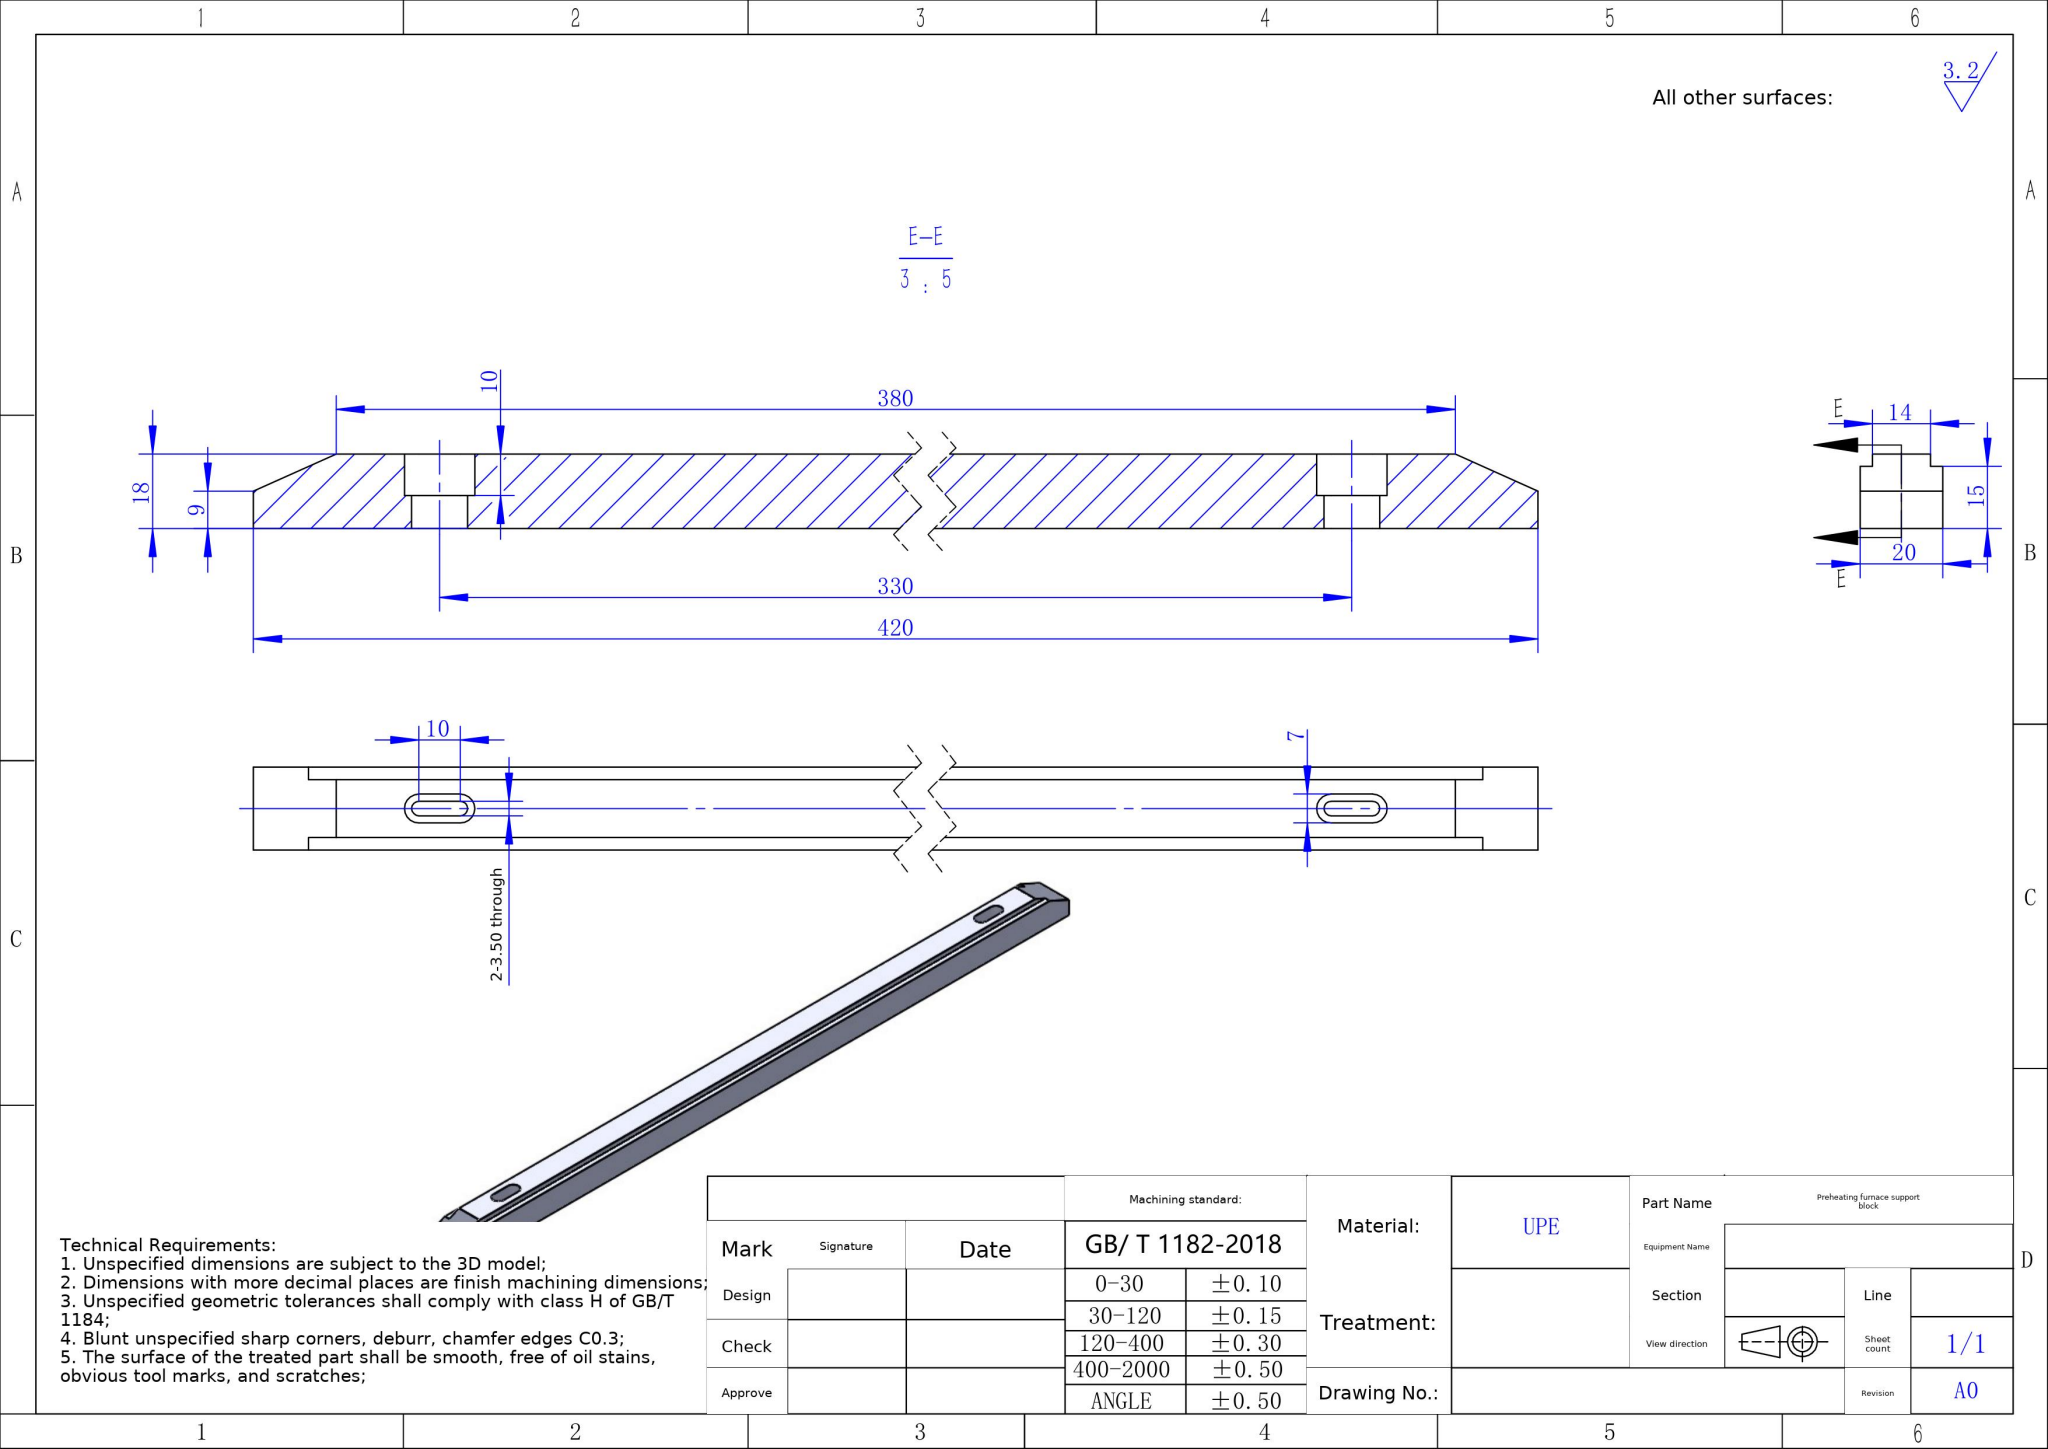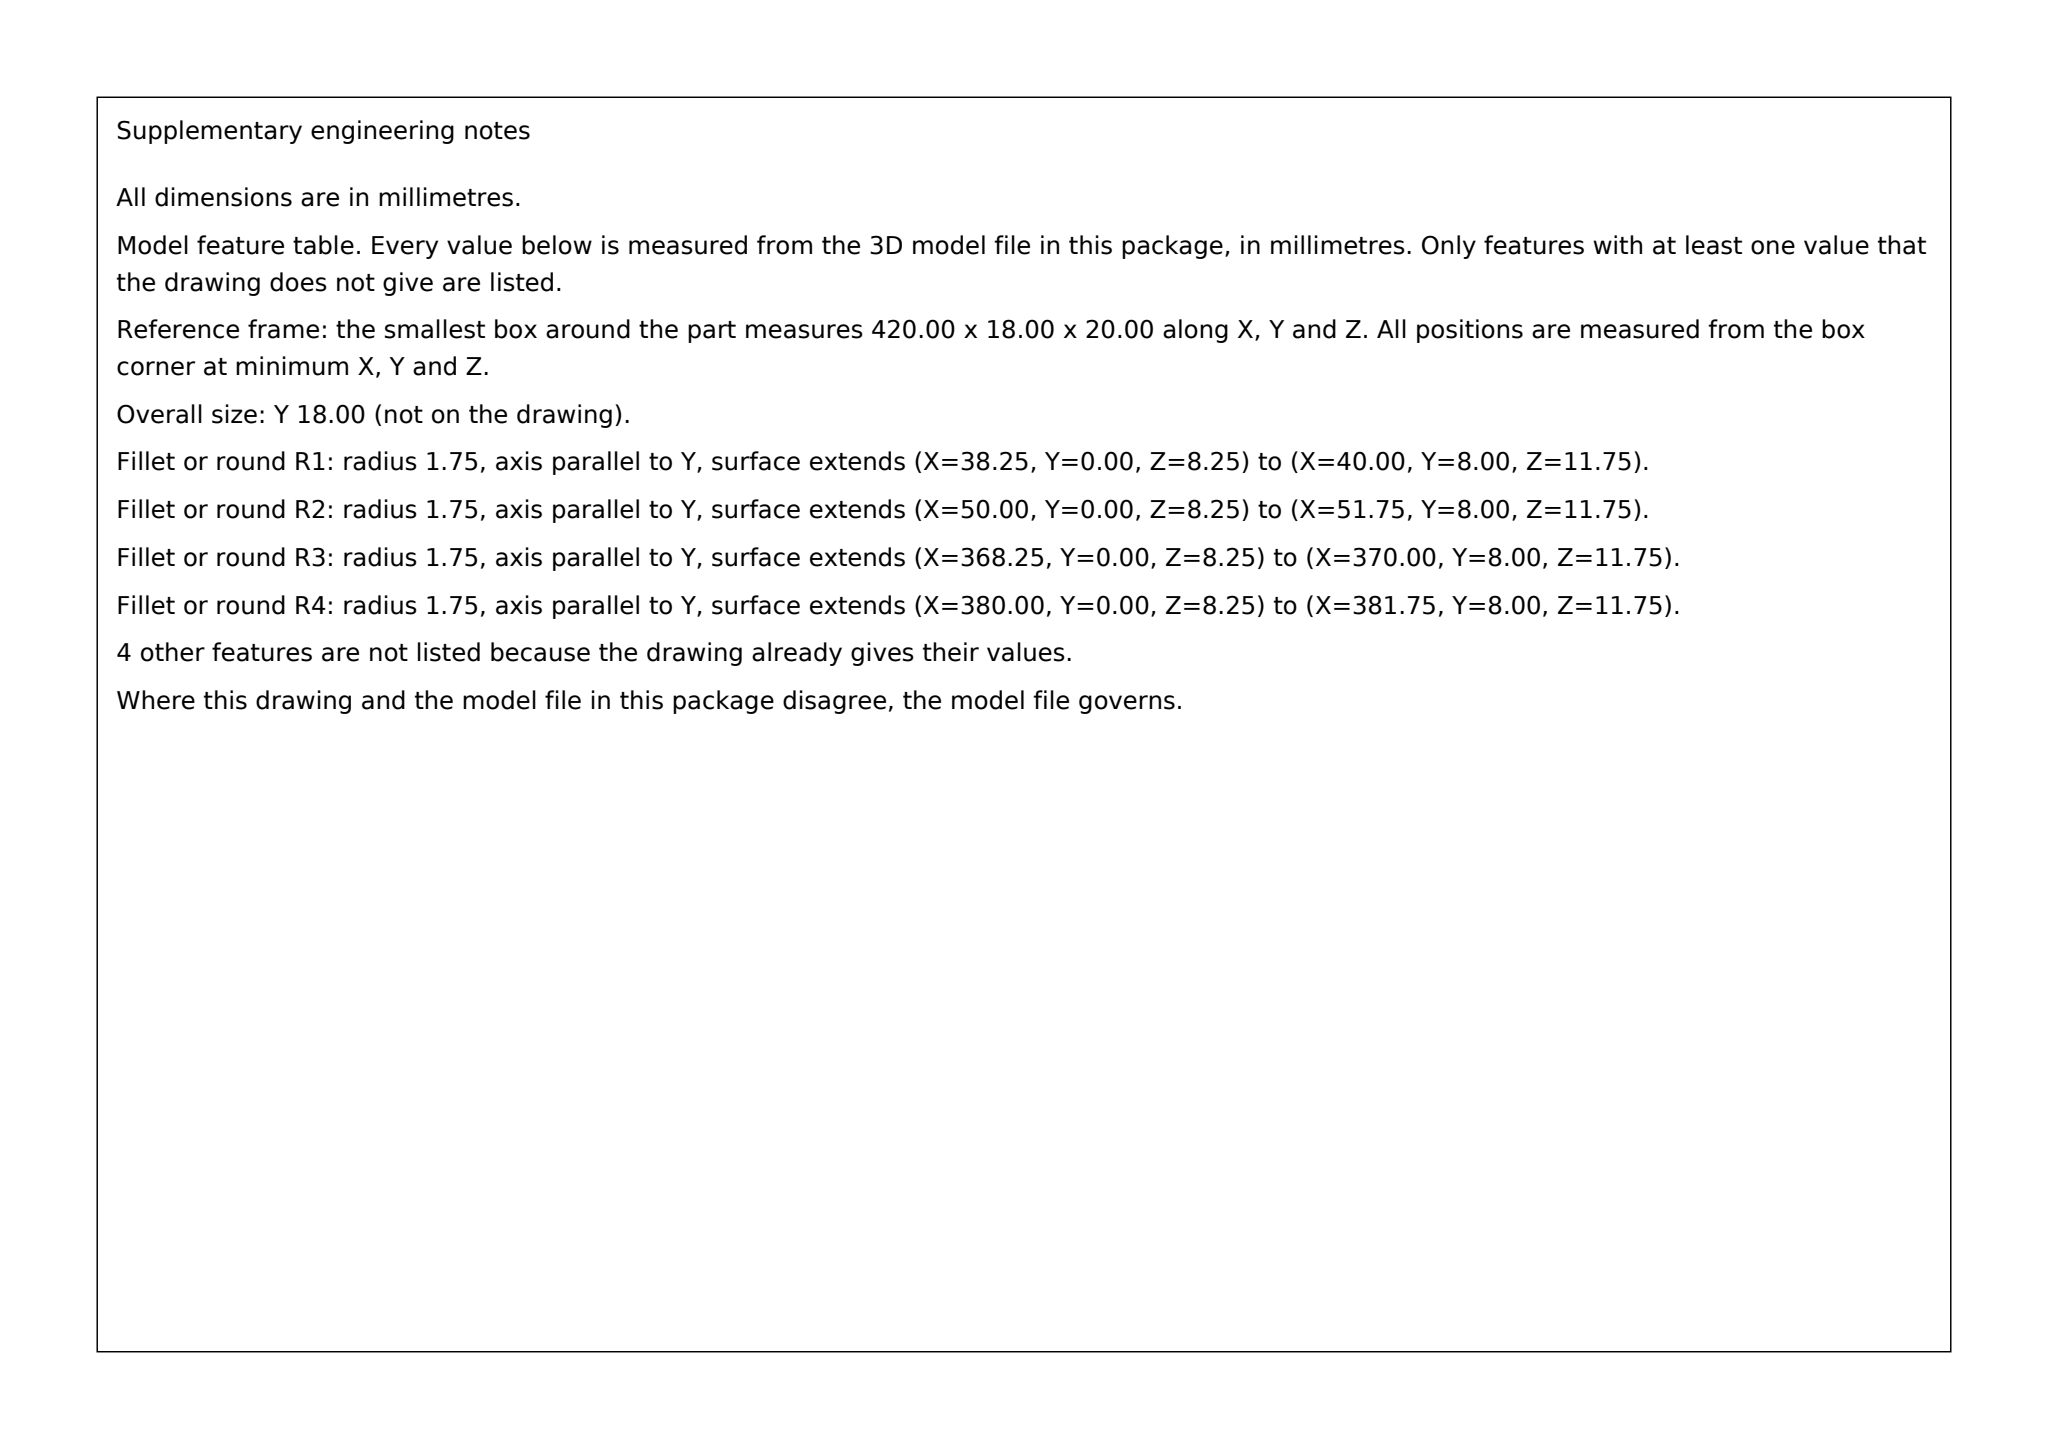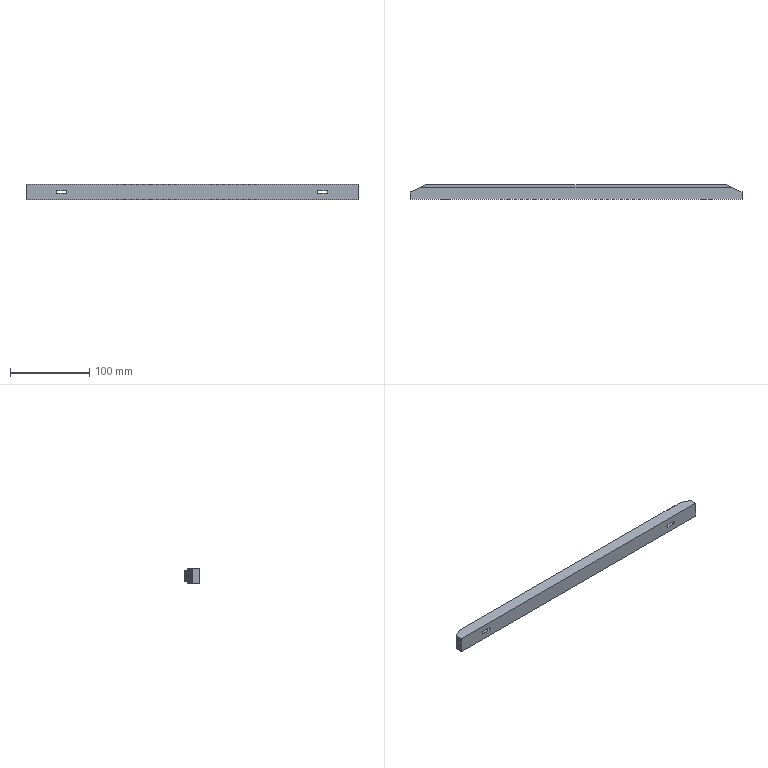Part | SolidWorks | mm | material UPE | 1 solid | 30 faces | box 420 x 18 x 20 mm | volume 137756 mm3 | plane 22 | cylinder 8 | commonest cylinder face diameters 3.5 x4 7 x4
build123d program:
from build123d import *

# Parameters (mm, degrees)
SKETCH1_W           = 420
SKETCH1_H           = 18
BOSS_EXTRUDE1_DEPTH = 10
CUT_EXTRUDE1_DEPTH  = 20
CUT_EXTRUDE2_DEPTH  = 212.007
SKETCH4_W           = 5.228
SKETCH4_H           = 5.603
CUT_EXTRUDE3_DEPTH  = 421.215
CUT_EXTRUDE4_DEPTH  = 10


with BuildPart() as part:
    # Sketch1 → Boss-Extrude1 (new, symmetric)
    with BuildSketch(Plane.XY):
        Rectangle(SKETCH1_W, SKETCH1_H)
    extrude(amount=BOSS_EXTRUDE1_DEPTH, both=True)

    # Sketch2 → Cut-Extrude1 (cut)
    with BuildSketch(Plane.XY.offset(10)):
        Polygon((210, 0), (190, 9), (210, 9), align=None)
        Polygon((-190, 9), (-210, 9), (-210, 0), align=None)
    extrude(amount=-CUT_EXTRUDE1_DEPTH, mode=Mode.SUBTRACT)

    # Sketch3 → Cut-Extrude2 (cut, through all)
    with BuildSketch(Plane(origin=(0, 9, 0), x_dir=(1, 0, 0), z_dir=(0, 1, 0))):
        with BuildLine():
            Line((160, 1.75), (170, 1.75))
            ThreePointArc((170, 1.75), (171.75, 0), (170, -1.75))
            Line((170, -1.75), (160, -1.75))
            ThreePointArc((160, -1.75), (158.25, 0), (160, 1.75))
        make_face()
        with BuildLine():
            Line((-160, 1.75), (-170, 1.75))
            ThreePointArc((-170, 1.75), (-171.75, 0), (-170, -1.75))
            Line((-170, -1.75), (-160, -1.75))
            ThreePointArc((-160, -1.75), (-158.25, 0), (-160, 1.75))
        make_face()
    extrude(amount=-CUT_EXTRUDE2_DEPTH, mode=Mode.SUBTRACT)

    # Sketch4 → Cut-Extrude3 (cut, through all)
    with BuildSketch(Plane(origin=(210, 0, 0), x_dir=(0, 0, -1), z_dir=(1, 0, 0))):
        with Locations((-9.614, 8.801)):
            Rectangle(SKETCH4_W, SKETCH4_H)
        with Locations((9.614, 8.801)):
            Rectangle(SKETCH4_W, SKETCH4_H)
    extrude(amount=-CUT_EXTRUDE3_DEPTH, mode=Mode.SUBTRACT)

    # Sketch5 → Cut-Extrude4 (cut)
    with BuildSketch(Plane(origin=(0, 9, 0), x_dir=(1, 0, 0), z_dir=(0, 1, 0))):
        with BuildLine():
            Line((160, -3.5), (170, -3.5))
            ThreePointArc((170, -3.5), (173.5, 0), (170, 3.5))
            Line((170, 3.5), (160, 3.5))
            ThreePointArc((160, 3.5), (156.5, 0), (160, -3.5))
        make_face()
        with BuildLine():
            Line((-170, 3.5), (-160, 3.5))
            ThreePointArc((-160, 3.5), (-156.5, 0), (-160, -3.5))
            Line((-160, -3.5), (-170, -3.5))
            ThreePointArc((-170, -3.5), (-173.5, 0), (-170, 3.5))
        make_face()
    extrude(amount=-CUT_EXTRUDE4_DEPTH, mode=Mode.SUBTRACT)


solid = part.part
STEP:
#1=CARTESIAN_POINT('',(160.,-1.,1.75));
#2=VERTEX_POINT('',#1);
#3=CARTESIAN_POINT('',(160.,-1.,-1.75));
#4=VERTEX_POINT('',#3);
#5=CARTESIAN_POINT('',(160.,-1.,-0.));
#6=DIRECTION('',(0.,-1.,0.));
#7=DIRECTION('',(0.,0.,1.));
#8=AXIS2_PLACEMENT_3D('',#5,#6,#7);
#9=CIRCLE('',#8,1.75);
#10=EDGE_CURVE('',#2,#4,#9,.T.);
#11=ORIENTED_EDGE('',*,*,#10,.F.);
#12=CARTESIAN_POINT('',(160.,-9.,1.75));
#13=VERTEX_POINT('',#12);
#14=CARTESIAN_POINT('',(160.,-9.,1.75));
#15=DIRECTION('',(0.,1.,0.));
#16=VECTOR('',#15,1000.);
#17=LINE('',#14,#16);
#18=EDGE_CURVE('',#13,#2,#17,.T.);
#19=ORIENTED_EDGE('',*,*,#18,.F.);
#20=CARTESIAN_POINT('',(160.,-9.,-1.75));
#21=VERTEX_POINT('',#20);
#22=CARTESIAN_POINT('',(160.,-9.,-0.));
#23=DIRECTION('',(0.,1.,0.));
#24=DIRECTION('',(0.,0.,1.));
#25=AXIS2_PLACEMENT_3D('',#22,#23,#24);
#26=CIRCLE('',#25,1.75);
#27=EDGE_CURVE('',#21,#13,#26,.T.);
#28=ORIENTED_EDGE('',*,*,#27,.F.);
#29=CARTESIAN_POINT('',(160.,-9.,-1.75));
#30=DIRECTION('',(0.,1.,0.));
#31=VECTOR('',#30,1000.);
#32=LINE('',#29,#31);
#33=EDGE_CURVE('',#21,#4,#32,.T.);
#34=ORIENTED_EDGE('',*,*,#33,.T.);
#35=EDGE_LOOP('',(#11,#19,#28,#34));
#36=FACE_OUTER_BOUND('',#35,.T.);
#37=CARTESIAN_POINT('',(160.,-9.,-0.));
#38=DIRECTION('',(0.,1.,0.));
#39=DIRECTION('',(0.,0.,1.));
#40=AXIS2_PLACEMENT_3D('',#37,#38,#39);
#41=CYLINDRICAL_SURFACE('',#40,1.75);
#42=ADVANCED_FACE('',(#36),#41,.F.);
#43=CARTESIAN_POINT('',(170.,-1.,-1.75));
#44=VERTEX_POINT('',#43);
#45=CARTESIAN_POINT('',(160.,-1.,-1.75));
#46=DIRECTION('',(1.,0.,-0.));
#47=VECTOR('',#46,1000.);
#48=LINE('',#45,#47);
#49=EDGE_CURVE('',#4,#44,#48,.T.);
#50=ORIENTED_EDGE('',*,*,#49,.F.);
#51=ORIENTED_EDGE('',*,*,#33,.F.);
#52=CARTESIAN_POINT('',(170.,-9.,-1.75));
#53=VERTEX_POINT('',#52);
#54=CARTESIAN_POINT('',(160.,-9.,-1.75));
#55=DIRECTION('',(-1.,0.,0.));
#56=VECTOR('',#55,1000.);
#57=LINE('',#54,#56);
#58=EDGE_CURVE('',#53,#21,#57,.T.);
#59=ORIENTED_EDGE('',*,*,#58,.F.);
#60=CARTESIAN_POINT('',(170.,-9.,-1.75));
#61=DIRECTION('',(0.,1.,0.));
#62=VECTOR('',#61,1000.);
#63=LINE('',#60,#62);
#64=EDGE_CURVE('',#53,#44,#63,.T.);
#65=ORIENTED_EDGE('',*,*,#64,.T.);
#66=EDGE_LOOP('',(#50,#51,#59,#65));
#67=FACE_OUTER_BOUND('',#66,.T.);
#68=CARTESIAN_POINT('',(160.,-9.,-1.75));
#69=DIRECTION('',(-0.,0.,-1.));
#70=DIRECTION('',(-1.,0.,0.));
#71=AXIS2_PLACEMENT_3D('',#68,#69,#70);
#72=PLANE('',#71);
#73=ADVANCED_FACE('',(#67),#72,.F.);
#74=CARTESIAN_POINT('',(170.,-1.,1.75));
#75=VERTEX_POINT('',#74);
#76=CARTESIAN_POINT('',(170.,-1.,-0.));
#77=DIRECTION('',(0.,-1.,0.));
#78=DIRECTION('',(0.,0.,1.));
#79=AXIS2_PLACEMENT_3D('',#76,#77,#78);
#80=CIRCLE('',#79,1.75);
#81=EDGE_CURVE('',#44,#75,#80,.T.);
#82=ORIENTED_EDGE('',*,*,#81,.F.);
#83=ORIENTED_EDGE('',*,*,#64,.F.);
#84=CARTESIAN_POINT('',(170.,-9.,1.75));
#85=VERTEX_POINT('',#84);
#86=CARTESIAN_POINT('',(170.,-9.,-0.));
#87=DIRECTION('',(0.,1.,0.));
#88=DIRECTION('',(0.,0.,1.));
#89=AXIS2_PLACEMENT_3D('',#86,#87,#88);
#90=CIRCLE('',#89,1.75);
#91=EDGE_CURVE('',#85,#53,#90,.T.);
#92=ORIENTED_EDGE('',*,*,#91,.F.);
#93=CARTESIAN_POINT('',(170.,-9.,1.75));
#94=DIRECTION('',(0.,1.,0.));
#95=VECTOR('',#94,1000.);
#96=LINE('',#93,#95);
#97=EDGE_CURVE('',#85,#75,#96,.T.);
#98=ORIENTED_EDGE('',*,*,#97,.T.);
#99=EDGE_LOOP('',(#82,#83,#92,#98));
#100=FACE_OUTER_BOUND('',#99,.T.);
#101=CARTESIAN_POINT('',(170.,-9.,-0.));
#102=DIRECTION('',(0.,1.,0.));
#103=DIRECTION('',(0.,0.,1.));
#104=AXIS2_PLACEMENT_3D('',#101,#102,#103);
#105=CYLINDRICAL_SURFACE('',#104,1.75);
#106=ADVANCED_FACE('',(#100),#105,.F.);
#107=CARTESIAN_POINT('',(160.,-1.,1.75));
#108=DIRECTION('',(-1.,0.,0.));
#109=VECTOR('',#108,1000.);
#110=LINE('',#107,#109);
#111=EDGE_CURVE('',#75,#2,#110,.T.);
#112=ORIENTED_EDGE('',*,*,#111,.F.);
#113=ORIENTED_EDGE('',*,*,#97,.F.);
#114=CARTESIAN_POINT('',(160.,-9.,1.75));
#115=DIRECTION('',(1.,0.,0.));
#116=VECTOR('',#115,1000.);
#117=LINE('',#114,#116);
#118=EDGE_CURVE('',#13,#85,#117,.T.);
#119=ORIENTED_EDGE('',*,*,#118,.F.);
#120=ORIENTED_EDGE('',*,*,#18,.T.);
#121=EDGE_LOOP('',(#112,#113,#119,#120));
#122=FACE_OUTER_BOUND('',#121,.T.);
#123=CARTESIAN_POINT('',(160.,-9.,1.75));
#124=DIRECTION('',(0.,0.,1.));
#125=DIRECTION('',(1.,0.,0.));
#126=AXIS2_PLACEMENT_3D('',#123,#124,#125);
#127=PLANE('',#126);
#128=ADVANCED_FACE('',(#122),#127,.F.);
#129=CARTESIAN_POINT('',(210.,-9.,-10.));
#130=VERTEX_POINT('',#129);
#131=CARTESIAN_POINT('',(210.,-0.,-10.));
#132=VERTEX_POINT('',#131);
#133=CARTESIAN_POINT('',(210.,-9.,-10.));
#134=DIRECTION('',(0.,1.,0.));
#135=VECTOR('',#134,1000.);
#136=LINE('',#133,#135);
#137=EDGE_CURVE('',#130,#132,#136,.T.);
#138=ORIENTED_EDGE('',*,*,#137,.T.);
#139=CARTESIAN_POINT('',(210.,0.,10.));
#140=VERTEX_POINT('',#139);
#141=CARTESIAN_POINT('',(210.,0.,-10.));
#142=DIRECTION('',(0.,0.,1.));
#143=VECTOR('',#142,1000.);
#144=LINE('',#141,#143);
#145=EDGE_CURVE('',#132,#140,#144,.T.);
#146=ORIENTED_EDGE('',*,*,#145,.T.);
#147=CARTESIAN_POINT('',(210.,-9.,10.));
#148=VERTEX_POINT('',#147);
#149=CARTESIAN_POINT('',(210.,-9.,10.));
#150=DIRECTION('',(0.,1.,0.));
#151=VECTOR('',#150,1000.);
#152=LINE('',#149,#151);
#153=EDGE_CURVE('',#148,#140,#152,.T.);
#154=ORIENTED_EDGE('',*,*,#153,.F.);
#155=CARTESIAN_POINT('',(210.,-9.,10.));
#156=DIRECTION('',(0.,0.,-1.));
#157=VECTOR('',#156,1000.);
#158=LINE('',#155,#157);
#159=EDGE_CURVE('',#148,#130,#158,.T.);
#160=ORIENTED_EDGE('',*,*,#159,.T.);
#161=EDGE_LOOP('',(#138,#146,#154,#160));
#162=FACE_OUTER_BOUND('',#161,.T.);
#163=CARTESIAN_POINT('',(210.,-9.,10.));
#164=DIRECTION('',(-1.,0.,0.));
#165=DIRECTION('',(0.,0.,1.));
#166=AXIS2_PLACEMENT_3D('',#163,#164,#165);
#167=PLANE('',#166);
#168=ADVANCED_FACE('',(#162),#167,.F.);
#169=CARTESIAN_POINT('',(-160.,9.,-3.5));
#170=VERTEX_POINT('',#169);
#171=CARTESIAN_POINT('',(-170.,9.,-3.5));
#172=VERTEX_POINT('',#171);
#173=CARTESIAN_POINT('',(-170.,9.,-3.5));
#174=DIRECTION('',(-1.,0.,-0.));
#175=VECTOR('',#174,1000.);
#176=LINE('',#173,#175);
#177=EDGE_CURVE('',#170,#172,#176,.T.);
#178=ORIENTED_EDGE('',*,*,#177,.F.);
#179=CARTESIAN_POINT('',(-160.,9.,3.5));
#180=VERTEX_POINT('',#179);
#181=CARTESIAN_POINT('',(-160.,9.,-0.));
#182=DIRECTION('',(0.,1.,0.));
#183=DIRECTION('',(0.,0.,-1.));
#184=AXIS2_PLACEMENT_3D('',#181,#182,#183);
#185=CIRCLE('',#184,3.5);
#186=EDGE_CURVE('',#180,#170,#185,.T.);
#187=ORIENTED_EDGE('',*,*,#186,.F.);
#188=CARTESIAN_POINT('',(-170.,9.,3.5));
#189=VERTEX_POINT('',#188);
#190=CARTESIAN_POINT('',(-160.,9.,3.5));
#191=DIRECTION('',(1.,0.,0.));
#192=VECTOR('',#191,1000.);
#193=LINE('',#190,#192);
#194=EDGE_CURVE('',#189,#180,#193,.T.);
#195=ORIENTED_EDGE('',*,*,#194,.F.);
#196=CARTESIAN_POINT('',(-170.,9.,-0.));
#197=DIRECTION('',(0.,1.,0.));
#198=DIRECTION('',(0.,0.,-1.));
#199=AXIS2_PLACEMENT_3D('',#196,#197,#198);
#200=CIRCLE('',#199,3.5);
#201=EDGE_CURVE('',#172,#189,#200,.T.);
#202=ORIENTED_EDGE('',*,*,#201,.F.);
#203=EDGE_LOOP('',(#178,#187,#195,#202));
#204=FACE_BOUND('',#203,.T.);
#205=CARTESIAN_POINT('',(170.,9.,-3.5));
#206=VERTEX_POINT('',#205);
#207=CARTESIAN_POINT('',(160.,9.,-3.5));
#208=VERTEX_POINT('',#207);
#209=CARTESIAN_POINT('',(170.,9.,-3.5));
#210=DIRECTION('',(-1.,0.,0.));
#211=VECTOR('',#210,1000.);
#212=LINE('',#209,#211);
#213=EDGE_CURVE('',#206,#208,#212,.T.);
#214=ORIENTED_EDGE('',*,*,#213,.F.);
#215=CARTESIAN_POINT('',(170.,9.,3.5));
#216=VERTEX_POINT('',#215);
#217=CARTESIAN_POINT('',(170.,9.,-0.));
#218=DIRECTION('',(0.,1.,0.));
#219=DIRECTION('',(0.,0.,1.));
#220=AXIS2_PLACEMENT_3D('',#217,#218,#219);
#221=CIRCLE('',#220,3.5);
#222=EDGE_CURVE('',#216,#206,#221,.T.);
#223=ORIENTED_EDGE('',*,*,#222,.F.);
#224=CARTESIAN_POINT('',(160.,9.,3.5));
#225=VERTEX_POINT('',#224);
#226=CARTESIAN_POINT('',(160.,9.,3.5));
#227=DIRECTION('',(1.,0.,-0.));
#228=VECTOR('',#227,1000.);
#229=LINE('',#226,#228);
#230=EDGE_CURVE('',#225,#216,#229,.T.);
#231=ORIENTED_EDGE('',*,*,#230,.F.);
#232=CARTESIAN_POINT('',(160.,9.,-0.));
#233=DIRECTION('',(0.,1.,0.));
#234=DIRECTION('',(0.,0.,1.));
#235=AXIS2_PLACEMENT_3D('',#232,#233,#234);
#236=CIRCLE('',#235,3.5);
#237=EDGE_CURVE('',#208,#225,#236,.T.);
#238=ORIENTED_EDGE('',*,*,#237,.F.);
#239=EDGE_LOOP('',(#214,#223,#231,#238));
#240=FACE_BOUND('',#239,.T.);
#241=CARTESIAN_POINT('',(-190.,9.,-7.));
#242=VERTEX_POINT('',#241);
#243=CARTESIAN_POINT('',(-190.,9.,7.));
#244=VERTEX_POINT('',#243);
#245=CARTESIAN_POINT('',(-190.,9.,-10.));
#246=DIRECTION('',(0.,0.,1.));
#247=VECTOR('',#246,1000.);
#248=LINE('',#245,#247);
#249=EDGE_CURVE('',#242,#244,#248,.T.);
#250=ORIENTED_EDGE('',*,*,#249,.T.);
#251=CARTESIAN_POINT('',(190.,9.,7.));
#252=VERTEX_POINT('',#251);
#253=CARTESIAN_POINT('',(-210.,9.,7.));
#254=DIRECTION('',(1.,0.,0.));
#255=VECTOR('',#254,1000.);
#256=LINE('',#253,#255);
#257=EDGE_CURVE('',#244,#252,#256,.T.);
#258=ORIENTED_EDGE('',*,*,#257,.T.);
#259=CARTESIAN_POINT('',(190.,9.,-7.));
#260=VERTEX_POINT('',#259);
#261=CARTESIAN_POINT('',(190.,9.,-10.));
#262=DIRECTION('',(0.,0.,1.));
#263=VECTOR('',#262,1000.);
#264=LINE('',#261,#263);
#265=EDGE_CURVE('',#260,#252,#264,.T.);
#266=ORIENTED_EDGE('',*,*,#265,.F.);
#267=CARTESIAN_POINT('',(-210.,9.,-7.));
#268=DIRECTION('',(-1.,0.,0.));
#269=VECTOR('',#268,1000.);
#270=LINE('',#267,#269);
#271=EDGE_CURVE('',#260,#242,#270,.T.);
#272=ORIENTED_EDGE('',*,*,#271,.T.);
#273=EDGE_LOOP('',(#250,#258,#266,#272));
#274=FACE_OUTER_BOUND('',#273,.T.);
#275=CARTESIAN_POINT('',(-210.,9.,10.));
#276=DIRECTION('',(0.,-1.,0.));
#277=DIRECTION('',(0.,0.,-1.));
#278=AXIS2_PLACEMENT_3D('',#275,#276,#277);
#279=PLANE('',#278);
#280=ADVANCED_FACE('',(#204,#240,#274),#279,.F.);
#281=CARTESIAN_POINT('',(-210.,0.,10.));
#282=VERTEX_POINT('',#281);
#283=CARTESIAN_POINT('',(-210.,-9.,10.));
#284=VERTEX_POINT('',#283);
#285=CARTESIAN_POINT('',(-210.,-9.,10.));
#286=DIRECTION('',(0.,-1.,0.));
#287=VECTOR('',#286,1000.);
#288=LINE('',#285,#287);
#289=EDGE_CURVE('',#282,#284,#288,.T.);
#290=ORIENTED_EDGE('',*,*,#289,.F.);
#291=CARTESIAN_POINT('',(-210.,0.,-10.));
#292=VERTEX_POINT('',#291);
#293=CARTESIAN_POINT('',(-210.,0.,-10.));
#294=DIRECTION('',(0.,0.,1.));
#295=VECTOR('',#294,1000.);
#296=LINE('',#293,#295);
#297=EDGE_CURVE('',#292,#282,#296,.T.);
#298=ORIENTED_EDGE('',*,*,#297,.F.);
#299=CARTESIAN_POINT('',(-210.,-9.,-10.));
#300=VERTEX_POINT('',#299);
#301=CARTESIAN_POINT('',(-210.,-9.,-10.));
#302=DIRECTION('',(0.,-1.,0.));
#303=VECTOR('',#302,1000.);
#304=LINE('',#301,#303);
#305=EDGE_CURVE('',#292,#300,#304,.T.);
#306=ORIENTED_EDGE('',*,*,#305,.T.);
#307=CARTESIAN_POINT('',(-210.,-9.,10.));
#308=DIRECTION('',(0.,0.,-1.));
#309=VECTOR('',#308,1000.);
#310=LINE('',#307,#309);
#311=EDGE_CURVE('',#284,#300,#310,.T.);
#312=ORIENTED_EDGE('',*,*,#311,.F.);
#313=EDGE_LOOP('',(#290,#298,#306,#312));
#314=FACE_OUTER_BOUND('',#313,.T.);
#315=CARTESIAN_POINT('',(-210.,-9.,10.));
#316=DIRECTION('',(1.,0.,0.));
#317=DIRECTION('',(0.,0.,-1.));
#318=AXIS2_PLACEMENT_3D('',#315,#316,#317);
#319=PLANE('',#318);
#320=ADVANCED_FACE('',(#314),#319,.F.);
#321=ORIENTED_EDGE('',*,*,#58,.T.);
#322=ORIENTED_EDGE('',*,*,#27,.T.);
#323=ORIENTED_EDGE('',*,*,#118,.T.);
#324=ORIENTED_EDGE('',*,*,#91,.T.);
#325=EDGE_LOOP('',(#321,#322,#323,#324));
#326=FACE_BOUND('',#325,.T.);
#327=CARTESIAN_POINT('',(-170.,-9.,1.75));
#328=VERTEX_POINT('',#327);
#329=CARTESIAN_POINT('',(-160.,-9.,1.75));
#330=VERTEX_POINT('',#329);
#331=CARTESIAN_POINT('',(-160.,-9.,1.75));
#332=DIRECTION('',(1.,0.,0.));
#333=VECTOR('',#332,1000.);
#334=LINE('',#331,#333);
#335=EDGE_CURVE('',#328,#330,#334,.T.);
#336=ORIENTED_EDGE('',*,*,#335,.T.);
#337=CARTESIAN_POINT('',(-160.,-9.,-1.75));
#338=VERTEX_POINT('',#337);
#339=CARTESIAN_POINT('',(-160.,-9.,-0.));
#340=DIRECTION('',(0.,1.,0.));
#341=DIRECTION('',(0.,0.,-1.));
#342=AXIS2_PLACEMENT_3D('',#339,#340,#341);
#343=CIRCLE('',#342,1.75);
#344=EDGE_CURVE('',#330,#338,#343,.T.);
#345=ORIENTED_EDGE('',*,*,#344,.T.);
#346=CARTESIAN_POINT('',(-170.,-9.,-1.75));
#347=VERTEX_POINT('',#346);
#348=CARTESIAN_POINT('',(-160.,-9.,-1.75));
#349=DIRECTION('',(-1.,0.,-0.));
#350=VECTOR('',#349,1000.);
#351=LINE('',#348,#350);
#352=EDGE_CURVE('',#338,#347,#351,.T.);
#353=ORIENTED_EDGE('',*,*,#352,.T.);
#354=CARTESIAN_POINT('',(-170.,-9.,-0.));
#355=DIRECTION('',(0.,1.,0.));
#356=DIRECTION('',(0.,0.,-1.));
#357=AXIS2_PLACEMENT_3D('',#354,#355,#356);
#358=CIRCLE('',#357,1.75);
#359=EDGE_CURVE('',#347,#328,#358,.T.);
#360=ORIENTED_EDGE('',*,*,#359,.T.);
#361=EDGE_LOOP('',(#336,#345,#353,#360));
#362=FACE_BOUND('',#361,.T.);
#363=CARTESIAN_POINT('',(-210.,-9.,-10.));
#364=DIRECTION('',(1.,0.,0.));
#365=VECTOR('',#364,1000.);
#366=LINE('',#363,#365);
#367=EDGE_CURVE('',#300,#130,#366,.T.);
#368=ORIENTED_EDGE('',*,*,#367,.T.);
#369=ORIENTED_EDGE('',*,*,#159,.F.);
#370=CARTESIAN_POINT('',(-210.,-9.,10.));
#371=DIRECTION('',(1.,0.,0.));
#372=VECTOR('',#371,1000.);
#373=LINE('',#370,#372);
#374=EDGE_CURVE('',#284,#148,#373,.T.);
#375=ORIENTED_EDGE('',*,*,#374,.F.);
#376=ORIENTED_EDGE('',*,*,#311,.T.);
#377=EDGE_LOOP('',(#368,#369,#375,#376));
#378=FACE_OUTER_BOUND('',#377,.T.);
#379=CARTESIAN_POINT('',(-210.,-9.,10.));
#380=DIRECTION('',(0.,1.,0.));
#381=DIRECTION('',(0.,0.,1.));
#382=AXIS2_PLACEMENT_3D('',#379,#380,#381);
#383=PLANE('',#382);
#384=ADVANCED_FACE('',(#326,#362,#378),#383,.F.);
#385=CARTESIAN_POINT('',(196.667,6.,10.));
#386=VERTEX_POINT('',#385);
#387=CARTESIAN_POINT('',(210.,0.,10.));
#388=DIRECTION('',(0.9119,-0.4104,0.));
#389=VECTOR('',#388,1000.);
#390=LINE('',#387,#389);
#391=EDGE_CURVE('',#386,#140,#390,.T.);
#392=ORIENTED_EDGE('',*,*,#391,.F.);
#393=CARTESIAN_POINT('',(-196.667,6.,10.));
#394=VERTEX_POINT('',#393);
#395=CARTESIAN_POINT('',(0.,6.,10.));
#396=DIRECTION('',(-1.,0.,0.));
#397=VECTOR('',#396,1000.);
#398=LINE('',#395,#397);
#399=EDGE_CURVE('',#386,#394,#398,.T.);
#400=ORIENTED_EDGE('',*,*,#399,.T.);
#401=CARTESIAN_POINT('',(-210.,0.,10.));
#402=DIRECTION('',(0.9119,0.4104,0.));
#403=VECTOR('',#402,1000.);
#404=LINE('',#401,#403);
#405=EDGE_CURVE('',#282,#394,#404,.T.);
#406=ORIENTED_EDGE('',*,*,#405,.F.);
#407=ORIENTED_EDGE('',*,*,#289,.T.);
#408=ORIENTED_EDGE('',*,*,#374,.T.);
#409=ORIENTED_EDGE('',*,*,#153,.T.);
#410=EDGE_LOOP('',(#392,#400,#406,#407,#408,#409));
#411=FACE_OUTER_BOUND('',#410,.T.);
#412=CARTESIAN_POINT('',(0.,0.,10.));
#413=DIRECTION('',(0.,0.,-1.));
#414=DIRECTION('',(-1.,0.,0.));
#415=AXIS2_PLACEMENT_3D('',#412,#413,#414);
#416=PLANE('',#415);
#417=ADVANCED_FACE('',(#411),#416,.F.);
#418=CARTESIAN_POINT('',(196.667,6.,-10.));
#419=VERTEX_POINT('',#418);
#420=CARTESIAN_POINT('',(-196.667,6.,-10.));
#421=VERTEX_POINT('',#420);
#422=CARTESIAN_POINT('',(0.,6.,-10.));
#423=DIRECTION('',(-1.,0.,0.));
#424=VECTOR('',#423,1000.);
#425=LINE('',#422,#424);
#426=EDGE_CURVE('',#419,#421,#425,.T.);
#427=ORIENTED_EDGE('',*,*,#426,.F.);
#428=CARTESIAN_POINT('',(210.,0.,-10.));
#429=DIRECTION('',(0.9119,-0.4104,0.));
#430=VECTOR('',#429,1000.);
#431=LINE('',#428,#430);
#432=EDGE_CURVE('',#419,#132,#431,.T.);
#433=ORIENTED_EDGE('',*,*,#432,.T.);
#434=ORIENTED_EDGE('',*,*,#137,.F.);
#435=ORIENTED_EDGE('',*,*,#367,.F.);
#436=ORIENTED_EDGE('',*,*,#305,.F.);
#437=CARTESIAN_POINT('',(-210.,0.,-10.));
#438=DIRECTION('',(0.9119,0.4104,0.));
#439=VECTOR('',#438,1000.);
#440=LINE('',#437,#439);
#441=EDGE_CURVE('',#292,#421,#440,.T.);
#442=ORIENTED_EDGE('',*,*,#441,.T.);
#443=EDGE_LOOP('',(#427,#433,#434,#435,#436,#442));
#444=FACE_OUTER_BOUND('',#443,.T.);
#445=CARTESIAN_POINT('',(0.,0.,-10.));
#446=DIRECTION('',(0.,0.,-1.));
#447=DIRECTION('',(-1.,0.,0.));
#448=AXIS2_PLACEMENT_3D('',#445,#446,#447);
#449=PLANE('',#448);
#450=ADVANCED_FACE('',(#444),#449,.T.);
#451=CARTESIAN_POINT('',(-196.667,6.,7.));
#452=VERTEX_POINT('',#451);
#453=CARTESIAN_POINT('',(-196.667,6.,-10.));
#454=DIRECTION('',(0.,0.,-1.));
#455=VECTOR('',#454,1000.);
#456=LINE('',#453,#455);
#457=EDGE_CURVE('',#394,#452,#456,.T.);
#458=ORIENTED_EDGE('',*,*,#457,.T.);
#459=CARTESIAN_POINT('',(-210.,0.,7.));
#460=DIRECTION('',(0.9119,0.4104,0.));
#461=VECTOR('',#460,1000.);
#462=LINE('',#459,#461);
#463=EDGE_CURVE('',#452,#244,#462,.T.);
#464=ORIENTED_EDGE('',*,*,#463,.T.);
#465=ORIENTED_EDGE('',*,*,#249,.F.);
#466=CARTESIAN_POINT('',(-196.667,6.,-7.));
#467=VERTEX_POINT('',#466);
#468=CARTESIAN_POINT('',(-210.,0.,-7.));
#469=DIRECTION('',(-0.9119,-0.4104,0.));
#470=VECTOR('',#469,1000.);
#471=LINE('',#468,#470);
#472=EDGE_CURVE('',#242,#467,#471,.T.);
#473=ORIENTED_EDGE('',*,*,#472,.T.);
#474=CARTESIAN_POINT('',(-196.667,6.,-10.));
#475=DIRECTION('',(0.,0.,-1.));
#476=VECTOR('',#475,1000.);
#477=LINE('',#474,#476);
#478=EDGE_CURVE('',#467,#421,#477,.T.);
#479=ORIENTED_EDGE('',*,*,#478,.T.);
#480=ORIENTED_EDGE('',*,*,#441,.F.);
#481=ORIENTED_EDGE('',*,*,#297,.T.);
#482=ORIENTED_EDGE('',*,*,#405,.T.);
#483=EDGE_LOOP('',(#458,#464,#465,#473,#479,#480,#481,#482));
#484=FACE_OUTER_BOUND('',#483,.T.);
#485=CARTESIAN_POINT('',(-210.,0.,-10.));
#486=DIRECTION('',(0.4104,-0.9119,0.));
#487=DIRECTION('',(0.9119,0.4104,0.));
#488=AXIS2_PLACEMENT_3D('',#485,#486,#487);
#489=PLANE('',#488);
#490=ADVANCED_FACE('',(#484),#489,.F.);
#491=ORIENTED_EDGE('',*,*,#265,.T.);
#492=CARTESIAN_POINT('',(196.667,6.,7.));
#493=VERTEX_POINT('',#492);
#494=CARTESIAN_POINT('',(210.,0.,7.));
#495=DIRECTION('',(0.9119,-0.4104,-0.));
#496=VECTOR('',#495,1000.);
#497=LINE('',#494,#496);
#498=EDGE_CURVE('',#252,#493,#497,.T.);
#499=ORIENTED_EDGE('',*,*,#498,.T.);
#500=CARTESIAN_POINT('',(196.667,6.,-10.));
#501=DIRECTION('',(0.,0.,1.));
#502=VECTOR('',#501,1000.);
#503=LINE('',#500,#502);
#504=EDGE_CURVE('',#493,#386,#503,.T.);
#505=ORIENTED_EDGE('',*,*,#504,.T.);
#506=ORIENTED_EDGE('',*,*,#391,.T.);
#507=ORIENTED_EDGE('',*,*,#145,.F.);
#508=ORIENTED_EDGE('',*,*,#432,.F.);
#509=CARTESIAN_POINT('',(196.667,6.,-7.));
#510=VERTEX_POINT('',#509);
#511=CARTESIAN_POINT('',(196.667,6.,-10.));
#512=DIRECTION('',(0.,0.,1.));
#513=VECTOR('',#512,1000.);
#514=LINE('',#511,#513);
#515=EDGE_CURVE('',#419,#510,#514,.T.);
#516=ORIENTED_EDGE('',*,*,#515,.T.);
#517=CARTESIAN_POINT('',(210.,0.,-7.));
#518=DIRECTION('',(-0.9119,0.4104,-0.));
#519=VECTOR('',#518,1000.);
#520=LINE('',#517,#519);
#521=EDGE_CURVE('',#510,#260,#520,.T.);
#522=ORIENTED_EDGE('',*,*,#521,.T.);
#523=EDGE_LOOP('',(#491,#499,#505,#506,#507,#508,#516,#522));
#524=FACE_OUTER_BOUND('',#523,.T.);
#525=CARTESIAN_POINT('',(210.,0.,-10.));
#526=DIRECTION('',(-0.4104,-0.9119,0.));
#527=DIRECTION('',(0.9119,-0.4104,0.));
#528=AXIS2_PLACEMENT_3D('',#525,#526,#527);
#529=PLANE('',#528);
#530=ADVANCED_FACE('',(#524),#529,.F.);
#531=CARTESIAN_POINT('',(-160.,-1.,1.75));
#532=VERTEX_POINT('',#531);
#533=CARTESIAN_POINT('',(-160.,-9.,1.75));
#534=DIRECTION('',(0.,1.,0.));
#535=VECTOR('',#534,1000.);
#536=LINE('',#533,#535);
#537=EDGE_CURVE('',#330,#532,#536,.T.);
#538=ORIENTED_EDGE('',*,*,#537,.T.);
#539=CARTESIAN_POINT('',(-160.,-1.,-1.75));
#540=VERTEX_POINT('',#539);
#541=CARTESIAN_POINT('',(-160.,-1.,-0.));
#542=DIRECTION('',(0.,1.,0.));
#543=DIRECTION('',(0.,0.,-1.));
#544=AXIS2_PLACEMENT_3D('',#541,#542,#543);
#545=CIRCLE('',#544,1.75);
#546=EDGE_CURVE('',#532,#540,#545,.T.);
#547=ORIENTED_EDGE('',*,*,#546,.T.);
#548=CARTESIAN_POINT('',(-160.,-9.,-1.75));
#549=DIRECTION('',(0.,1.,0.));
#550=VECTOR('',#549,1000.);
#551=LINE('',#548,#550);
#552=EDGE_CURVE('',#338,#540,#551,.T.);
#553=ORIENTED_EDGE('',*,*,#552,.F.);
#554=ORIENTED_EDGE('',*,*,#344,.F.);
#555=EDGE_LOOP('',(#538,#547,#553,#554));
#556=FACE_OUTER_BOUND('',#555,.T.);
#557=CARTESIAN_POINT('',(-160.,-9.,-0.));
#558=DIRECTION('',(0.,1.,0.));
#559=DIRECTION('',(0.,0.,1.));
#560=AXIS2_PLACEMENT_3D('',#557,#558,#559);
#561=CYLINDRICAL_SURFACE('',#560,1.75);
#562=ADVANCED_FACE('',(#556),#561,.F.);
#563=CARTESIAN_POINT('',(-170.,-1.,1.75));
#564=VERTEX_POINT('',#563);
#565=CARTESIAN_POINT('',(-170.,-9.,1.75));
#566=DIRECTION('',(0.,1.,0.));
#567=VECTOR('',#566,1000.);
#568=LINE('',#565,#567);
#569=EDGE_CURVE('',#328,#564,#568,.T.);
#570=ORIENTED_EDGE('',*,*,#569,.T.);
#571=CARTESIAN_POINT('',(-160.,-1.,1.75));
#572=DIRECTION('',(1.,0.,0.));
#573=VECTOR('',#572,1000.);
#574=LINE('',#571,#573);
#575=EDGE_CURVE('',#564,#532,#574,.T.);
#576=ORIENTED_EDGE('',*,*,#575,.T.);
#577=ORIENTED_EDGE('',*,*,#537,.F.);
#578=ORIENTED_EDGE('',*,*,#335,.F.);
#579=EDGE_LOOP('',(#570,#576,#577,#578));
#580=FACE_OUTER_BOUND('',#579,.T.);
#581=CARTESIAN_POINT('',(-160.,-9.,1.75));
#582=DIRECTION('',(0.,0.,1.));
#583=DIRECTION('',(1.,0.,0.));
#584=AXIS2_PLACEMENT_3D('',#581,#582,#583);
#585=PLANE('',#584);
#586=ADVANCED_FACE('',(#580),#585,.F.);
#587=CARTESIAN_POINT('',(-170.,-1.,-1.75));
#588=VERTEX_POINT('',#587);
#589=CARTESIAN_POINT('',(-170.,-9.,-1.75));
#590=DIRECTION('',(0.,1.,0.));
#591=VECTOR('',#590,1000.);
#592=LINE('',#589,#591);
#593=EDGE_CURVE('',#347,#588,#592,.T.);
#594=ORIENTED_EDGE('',*,*,#593,.T.);
#595=CARTESIAN_POINT('',(-170.,-1.,-0.));
#596=DIRECTION('',(0.,1.,0.));
#597=DIRECTION('',(0.,0.,-1.));
#598=AXIS2_PLACEMENT_3D('',#595,#596,#597);
#599=CIRCLE('',#598,1.75);
#600=EDGE_CURVE('',#588,#564,#599,.T.);
#601=ORIENTED_EDGE('',*,*,#600,.T.);
#602=ORIENTED_EDGE('',*,*,#569,.F.);
#603=ORIENTED_EDGE('',*,*,#359,.F.);
#604=EDGE_LOOP('',(#594,#601,#602,#603));
#605=FACE_OUTER_BOUND('',#604,.T.);
#606=CARTESIAN_POINT('',(-170.,-9.,-0.));
#607=DIRECTION('',(0.,1.,0.));
#608=DIRECTION('',(0.,0.,1.));
#609=AXIS2_PLACEMENT_3D('',#606,#607,#608);
#610=CYLINDRICAL_SURFACE('',#609,1.75);
#611=ADVANCED_FACE('',(#605),#610,.F.);
#612=ORIENTED_EDGE('',*,*,#552,.T.);
#613=CARTESIAN_POINT('',(-160.,-1.,-1.75));
#614=DIRECTION('',(-1.,0.,-0.));
#615=VECTOR('',#614,1000.);
#616=LINE('',#613,#615);
#617=EDGE_CURVE('',#540,#588,#616,.T.);
#618=ORIENTED_EDGE('',*,*,#617,.T.);
#619=ORIENTED_EDGE('',*,*,#593,.F.);
#620=ORIENTED_EDGE('',*,*,#352,.F.);
#621=EDGE_LOOP('',(#612,#618,#619,#620));
#622=FACE_OUTER_BOUND('',#621,.T.);
#623=CARTESIAN_POINT('',(-160.,-9.,-1.75));
#624=DIRECTION('',(0.,0.,-1.));
#625=DIRECTION('',(-1.,0.,-0.));
#626=AXIS2_PLACEMENT_3D('',#623,#624,#625);
#627=PLANE('',#626);
#628=ADVANCED_FACE('',(#622),#627,.F.);
#629=CARTESIAN_POINT('',(-210.,6.,-7.));
#630=DIRECTION('',(1.,0.,0.));
#631=VECTOR('',#630,1000.);
#632=LINE('',#629,#631);
#633=EDGE_CURVE('',#467,#510,#632,.T.);
#634=ORIENTED_EDGE('',*,*,#633,.T.);
#635=ORIENTED_EDGE('',*,*,#515,.F.);
#636=ORIENTED_EDGE('',*,*,#426,.T.);
#637=ORIENTED_EDGE('',*,*,#478,.F.);
#638=EDGE_LOOP('',(#634,#635,#636,#637));
#639=FACE_OUTER_BOUND('',#638,.T.);
#640=CARTESIAN_POINT('',(-210.,6.,-12.228));
#641=DIRECTION('',(0.,-1.,0.));
#642=DIRECTION('',(0.,0.,-1.));
#643=AXIS2_PLACEMENT_3D('',#640,#641,#642);
#644=PLANE('',#643);
#645=ADVANCED_FACE('',(#639),#644,.F.);
#646=ORIENTED_EDGE('',*,*,#271,.F.);
#647=ORIENTED_EDGE('',*,*,#521,.F.);
#648=ORIENTED_EDGE('',*,*,#633,.F.);
#649=ORIENTED_EDGE('',*,*,#472,.F.);
#650=EDGE_LOOP('',(#646,#647,#648,#649));
#651=FACE_OUTER_BOUND('',#650,.T.);
#652=CARTESIAN_POINT('',(-210.,11.603,-7.));
#653=DIRECTION('',(0.,0.,1.));
#654=DIRECTION('',(0.,-1.,0.));
#655=AXIS2_PLACEMENT_3D('',#652,#653,#654);
#656=PLANE('',#655);
#657=ADVANCED_FACE('',(#651),#656,.F.);
#658=CARTESIAN_POINT('',(-210.,6.,7.));
#659=DIRECTION('',(1.,0.,0.));
#660=VECTOR('',#659,1000.);
#661=LINE('',#658,#660);
#662=EDGE_CURVE('',#452,#493,#661,.T.);
#663=ORIENTED_EDGE('',*,*,#662,.T.);
#664=ORIENTED_EDGE('',*,*,#498,.F.);
#665=ORIENTED_EDGE('',*,*,#257,.F.);
#666=ORIENTED_EDGE('',*,*,#463,.F.);
#667=EDGE_LOOP('',(#663,#664,#665,#666));
#668=FACE_OUTER_BOUND('',#667,.T.);
#669=CARTESIAN_POINT('',(-210.,11.603,7.));
#670=DIRECTION('',(0.,0.,-1.));
#671=DIRECTION('',(0.,1.,0.));
#672=AXIS2_PLACEMENT_3D('',#669,#670,#671);
#673=PLANE('',#672);
#674=ADVANCED_FACE('',(#668),#673,.F.);
#675=ORIENTED_EDGE('',*,*,#399,.F.);
#676=ORIENTED_EDGE('',*,*,#504,.F.);
#677=ORIENTED_EDGE('',*,*,#662,.F.);
#678=ORIENTED_EDGE('',*,*,#457,.F.);
#679=EDGE_LOOP('',(#675,#676,#677,#678));
#680=FACE_OUTER_BOUND('',#679,.T.);
#681=CARTESIAN_POINT('',(-210.,6.,12.228));
#682=DIRECTION('',(0.,-1.,0.));
#683=DIRECTION('',(0.,0.,-1.));
#684=AXIS2_PLACEMENT_3D('',#681,#682,#683);
#685=PLANE('',#684);
#686=ADVANCED_FACE('',(#680),#685,.F.);
#687=CARTESIAN_POINT('',(170.,-1.,3.5));
#688=VERTEX_POINT('',#687);
#689=CARTESIAN_POINT('',(170.,-1.,-3.5));
#690=VERTEX_POINT('',#689);
#691=CARTESIAN_POINT('',(170.,-1.,-0.));
#692=DIRECTION('',(0.,1.,0.));
#693=DIRECTION('',(0.,0.,1.));
#694=AXIS2_PLACEMENT_3D('',#691,#692,#693);
#695=CIRCLE('',#694,3.5);
#696=EDGE_CURVE('',#688,#690,#695,.T.);
#697=ORIENTED_EDGE('',*,*,#696,.T.);
#698=CARTESIAN_POINT('',(160.,-1.,-3.5));
#699=VERTEX_POINT('',#698);
#700=CARTESIAN_POINT('',(170.,-1.,-3.5));
#701=DIRECTION('',(-1.,0.,0.));
#702=VECTOR('',#701,1000.);
#703=LINE('',#700,#702);
#704=EDGE_CURVE('',#690,#699,#703,.T.);
#705=ORIENTED_EDGE('',*,*,#704,.T.);
#706=CARTESIAN_POINT('',(160.,-1.,3.5));
#707=VERTEX_POINT('',#706);
#708=CARTESIAN_POINT('',(160.,-1.,-0.));
#709=DIRECTION('',(0.,1.,0.));
#710=DIRECTION('',(0.,0.,1.));
#711=AXIS2_PLACEMENT_3D('',#708,#709,#710);
#712=CIRCLE('',#711,3.5);
#713=EDGE_CURVE('',#699,#707,#712,.T.);
#714=ORIENTED_EDGE('',*,*,#713,.T.);
#715=CARTESIAN_POINT('',(160.,-1.,3.5));
#716=DIRECTION('',(1.,0.,-0.));
#717=VECTOR('',#716,1000.);
#718=LINE('',#715,#717);
#719=EDGE_CURVE('',#707,#688,#718,.T.);
#720=ORIENTED_EDGE('',*,*,#719,.T.);
#721=EDGE_LOOP('',(#697,#705,#714,#720));
#722=FACE_OUTER_BOUND('',#721,.T.);
#723=ORIENTED_EDGE('',*,*,#10,.T.);
#724=ORIENTED_EDGE('',*,*,#49,.T.);
#725=ORIENTED_EDGE('',*,*,#81,.T.);
#726=ORIENTED_EDGE('',*,*,#111,.T.);
#727=EDGE_LOOP('',(#723,#724,#725,#726));
#728=FACE_BOUND('',#727,.T.);
#729=CARTESIAN_POINT('',(170.,-1.,-0.));
#730=DIRECTION('',(0.,1.,0.));
#731=DIRECTION('',(0.,0.,1.));
#732=AXIS2_PLACEMENT_3D('',#729,#730,#731);
#733=PLANE('',#732);
#734=ADVANCED_FACE('',(#722,#728),#733,.T.);
#735=ORIENTED_EDGE('',*,*,#222,.T.);
#736=CARTESIAN_POINT('',(170.,-1.,-3.5));
#737=DIRECTION('',(0.,1.,0.));
#738=VECTOR('',#737,1000.);
#739=LINE('',#736,#738);
#740=EDGE_CURVE('',#690,#206,#739,.T.);
#741=ORIENTED_EDGE('',*,*,#740,.F.);
#742=ORIENTED_EDGE('',*,*,#696,.F.);
#743=CARTESIAN_POINT('',(170.,-1.,3.5));
#744=DIRECTION('',(0.,1.,0.));
#745=VECTOR('',#744,1000.);
#746=LINE('',#743,#745);
#747=EDGE_CURVE('',#688,#216,#746,.T.);
#748=ORIENTED_EDGE('',*,*,#747,.T.);
#749=EDGE_LOOP('',(#735,#741,#742,#748));
#750=FACE_OUTER_BOUND('',#749,.T.);
#751=CARTESIAN_POINT('',(170.,-1.,-0.));
#752=DIRECTION('',(0.,1.,0.));
#753=DIRECTION('',(0.,0.,1.));
#754=AXIS2_PLACEMENT_3D('',#751,#752,#753);
#755=CYLINDRICAL_SURFACE('',#754,3.5);
#756=ADVANCED_FACE('',(#750),#755,.F.);
#757=ORIENTED_EDGE('',*,*,#230,.T.);
#758=ORIENTED_EDGE('',*,*,#747,.F.);
#759=ORIENTED_EDGE('',*,*,#719,.F.);
#760=CARTESIAN_POINT('',(160.,-1.,3.5));
#761=DIRECTION('',(0.,1.,0.));
#762=VECTOR('',#761,1000.);
#763=LINE('',#760,#762);
#764=EDGE_CURVE('',#707,#225,#763,.T.);
#765=ORIENTED_EDGE('',*,*,#764,.T.);
#766=EDGE_LOOP('',(#757,#758,#759,#765));
#767=FACE_OUTER_BOUND('',#766,.T.);
#768=CARTESIAN_POINT('',(160.,-1.,3.5));
#769=DIRECTION('',(0.,0.,1.));
#770=DIRECTION('',(1.,0.,-0.));
#771=AXIS2_PLACEMENT_3D('',#768,#769,#770);
#772=PLANE('',#771);
#773=ADVANCED_FACE('',(#767),#772,.F.);
#774=ORIENTED_EDGE('',*,*,#237,.T.);
#775=ORIENTED_EDGE('',*,*,#764,.F.);
#776=ORIENTED_EDGE('',*,*,#713,.F.);
#777=CARTESIAN_POINT('',(160.,-1.,-3.5));
#778=DIRECTION('',(0.,1.,0.));
#779=VECTOR('',#778,1000.);
#780=LINE('',#777,#779);
#781=EDGE_CURVE('',#699,#208,#780,.T.);
#782=ORIENTED_EDGE('',*,*,#781,.T.);
#783=EDGE_LOOP('',(#774,#775,#776,#782));
#784=FACE_OUTER_BOUND('',#783,.T.);
#785=CARTESIAN_POINT('',(160.,-1.,-0.));
#786=DIRECTION('',(0.,1.,0.));
#787=DIRECTION('',(0.,0.,1.));
#788=AXIS2_PLACEMENT_3D('',#785,#786,#787);
#789=CYLINDRICAL_SURFACE('',#788,3.5);
#790=ADVANCED_FACE('',(#784),#789,.F.);
#791=ORIENTED_EDGE('',*,*,#213,.T.);
#792=ORIENTED_EDGE('',*,*,#781,.F.);
#793=ORIENTED_EDGE('',*,*,#704,.F.);
#794=ORIENTED_EDGE('',*,*,#740,.T.);
#795=EDGE_LOOP('',(#791,#792,#793,#794));
#796=FACE_OUTER_BOUND('',#795,.T.);
#797=CARTESIAN_POINT('',(170.,-1.,-3.5));
#798=DIRECTION('',(-0.,0.,-1.));
#799=DIRECTION('',(-1.,0.,0.));
#800=AXIS2_PLACEMENT_3D('',#797,#798,#799);
#801=PLANE('',#800);
#802=ADVANCED_FACE('',(#796),#801,.F.);
#803=CARTESIAN_POINT('',(-160.,-1.,3.5));
#804=VERTEX_POINT('',#803);
#805=CARTESIAN_POINT('',(-160.,-1.,-3.5));
#806=VERTEX_POINT('',#805);
#807=CARTESIAN_POINT('',(-160.,-1.,-0.));
#808=DIRECTION('',(0.,1.,0.));
#809=DIRECTION('',(0.,0.,-1.));
#810=AXIS2_PLACEMENT_3D('',#807,#808,#809);
#811=CIRCLE('',#810,3.5);
#812=EDGE_CURVE('',#804,#806,#811,.T.);
#813=ORIENTED_EDGE('',*,*,#812,.T.);
#814=CARTESIAN_POINT('',(-170.,-1.,-3.5));
#815=VERTEX_POINT('',#814);
#816=CARTESIAN_POINT('',(-170.,-1.,-3.5));
#817=DIRECTION('',(-1.,0.,-0.));
#818=VECTOR('',#817,1000.);
#819=LINE('',#816,#818);
#820=EDGE_CURVE('',#806,#815,#819,.T.);
#821=ORIENTED_EDGE('',*,*,#820,.T.);
#822=CARTESIAN_POINT('',(-170.,-1.,3.5));
#823=VERTEX_POINT('',#822);
#824=CARTESIAN_POINT('',(-170.,-1.,-0.));
#825=DIRECTION('',(0.,1.,0.));
#826=DIRECTION('',(0.,0.,-1.));
#827=AXIS2_PLACEMENT_3D('',#824,#825,#826);
#828=CIRCLE('',#827,3.5);
#829=EDGE_CURVE('',#815,#823,#828,.T.);
#830=ORIENTED_EDGE('',*,*,#829,.T.);
#831=CARTESIAN_POINT('',(-160.,-1.,3.5));
#832=DIRECTION('',(1.,0.,0.));
#833=VECTOR('',#832,1000.);
#834=LINE('',#831,#833);
#835=EDGE_CURVE('',#823,#804,#834,.T.);
#836=ORIENTED_EDGE('',*,*,#835,.T.);
#837=EDGE_LOOP('',(#813,#821,#830,#836));
#838=FACE_OUTER_BOUND('',#837,.T.);
#839=ORIENTED_EDGE('',*,*,#575,.F.);
#840=ORIENTED_EDGE('',*,*,#600,.F.);
#841=ORIENTED_EDGE('',*,*,#617,.F.);
#842=ORIENTED_EDGE('',*,*,#546,.F.);
#843=EDGE_LOOP('',(#839,#840,#841,#842));
#844=FACE_BOUND('',#843,.T.);
#845=CARTESIAN_POINT('',(-160.,-1.,-0.));
#846=DIRECTION('',(0.,-1.,0.));
#847=DIRECTION('',(0.,0.,-1.));
#848=AXIS2_PLACEMENT_3D('',#845,#846,#847);
#849=PLANE('',#848);
#850=ADVANCED_FACE('',(#838,#844),#849,.F.);
#851=ORIENTED_EDGE('',*,*,#186,.T.);
#852=CARTESIAN_POINT('',(-160.,-1.,-3.5));
#853=DIRECTION('',(0.,1.,0.));
#854=VECTOR('',#853,1000.);
#855=LINE('',#852,#854);
#856=EDGE_CURVE('',#806,#170,#855,.T.);
#857=ORIENTED_EDGE('',*,*,#856,.F.);
#858=ORIENTED_EDGE('',*,*,#812,.F.);
#859=CARTESIAN_POINT('',(-160.,-1.,3.5));
#860=DIRECTION('',(0.,1.,0.));
#861=VECTOR('',#860,1000.);
#862=LINE('',#859,#861);
#863=EDGE_CURVE('',#804,#180,#862,.T.);
#864=ORIENTED_EDGE('',*,*,#863,.T.);
#865=EDGE_LOOP('',(#851,#857,#858,#864));
#866=FACE_OUTER_BOUND('',#865,.T.);
#867=CARTESIAN_POINT('',(-160.,-1.,-0.));
#868=DIRECTION('',(0.,1.,0.));
#869=DIRECTION('',(0.,0.,1.));
#870=AXIS2_PLACEMENT_3D('',#867,#868,#869);
#871=CYLINDRICAL_SURFACE('',#870,3.5);
#872=ADVANCED_FACE('',(#866),#871,.F.);
#873=ORIENTED_EDGE('',*,*,#194,.T.);
#874=ORIENTED_EDGE('',*,*,#863,.F.);
#875=ORIENTED_EDGE('',*,*,#835,.F.);
#876=CARTESIAN_POINT('',(-170.,-1.,3.5));
#877=DIRECTION('',(0.,1.,0.));
#878=VECTOR('',#877,1000.);
#879=LINE('',#876,#878);
#880=EDGE_CURVE('',#823,#189,#879,.T.);
#881=ORIENTED_EDGE('',*,*,#880,.T.);
#882=EDGE_LOOP('',(#873,#874,#875,#881));
#883=FACE_OUTER_BOUND('',#882,.T.);
#884=CARTESIAN_POINT('',(-160.,-1.,3.5));
#885=DIRECTION('',(-0.,0.,1.));
#886=DIRECTION('',(1.,0.,0.));
#887=AXIS2_PLACEMENT_3D('',#884,#885,#886);
#888=PLANE('',#887);
#889=ADVANCED_FACE('',(#883),#888,.F.);
#890=ORIENTED_EDGE('',*,*,#201,.T.);
#891=ORIENTED_EDGE('',*,*,#880,.F.);
#892=ORIENTED_EDGE('',*,*,#829,.F.);
#893=CARTESIAN_POINT('',(-170.,-1.,-3.5));
#894=DIRECTION('',(0.,1.,0.));
#895=VECTOR('',#894,1000.);
#896=LINE('',#893,#895);
#897=EDGE_CURVE('',#815,#172,#896,.T.);
#898=ORIENTED_EDGE('',*,*,#897,.T.);
#899=EDGE_LOOP('',(#890,#891,#892,#898));
#900=FACE_OUTER_BOUND('',#899,.T.);
#901=CARTESIAN_POINT('',(-170.,-1.,-0.));
#902=DIRECTION('',(0.,1.,0.));
#903=DIRECTION('',(0.,0.,1.));
#904=AXIS2_PLACEMENT_3D('',#901,#902,#903);
#905=CYLINDRICAL_SURFACE('',#904,3.5);
#906=ADVANCED_FACE('',(#900),#905,.F.);
#907=ORIENTED_EDGE('',*,*,#177,.T.);
#908=ORIENTED_EDGE('',*,*,#897,.F.);
#909=ORIENTED_EDGE('',*,*,#820,.F.);
#910=ORIENTED_EDGE('',*,*,#856,.T.);
#911=EDGE_LOOP('',(#907,#908,#909,#910));
#912=FACE_OUTER_BOUND('',#911,.T.);
#913=CARTESIAN_POINT('',(-170.,-1.,-3.5));
#914=DIRECTION('',(0.,0.,-1.));
#915=DIRECTION('',(-1.,0.,-0.));
#916=AXIS2_PLACEMENT_3D('',#913,#914,#915);
#917=PLANE('',#916);
#918=ADVANCED_FACE('',(#912),#917,.F.);
#919=CLOSED_SHELL('',(#42,#73,#106,#128,#168,#280,#320,#384,#417,#450,#490,#530,#562,#586,#611,#628,#645,#657,#674,#686,#734,#756,#773,#790,#802,#850,#872,#889,#906,#918));
#920=MANIFOLD_SOLID_BREP('',#919);
#921=CARTESIAN_POINT('',(0.,0.,0.));
#922=DIRECTION('',(0.,0.,1.));
#923=DIRECTION('',(1.,0.,0.));
#924=AXIS2_PLACEMENT_3D('',#921,#922,#923);
#925=(LENGTH_UNIT()NAMED_UNIT(*)SI_UNIT(.MILLI.,.METRE.));
#926=UNCERTAINTY_MEASURE_WITH_UNIT(LENGTH_MEASURE(0.00001),#925,'','');
#927=(NAMED_UNIT(*)PLANE_ANGLE_UNIT()SI_UNIT($,.RADIAN.));
#928=(NAMED_UNIT(*)SI_UNIT($,.STERADIAN.)SOLID_ANGLE_UNIT());
#929=(GEOMETRIC_REPRESENTATION_CONTEXT(3)GLOBAL_UNCERTAINTY_ASSIGNED_CONTEXT((#926))GLOBAL_UNIT_ASSIGNED_CONTEXT((#925,#927,#928))REPRESENTATION_CONTEXT('',''));
#930=ADVANCED_BREP_SHAPE_REPRESENTATION('',(#920,#924),#929);